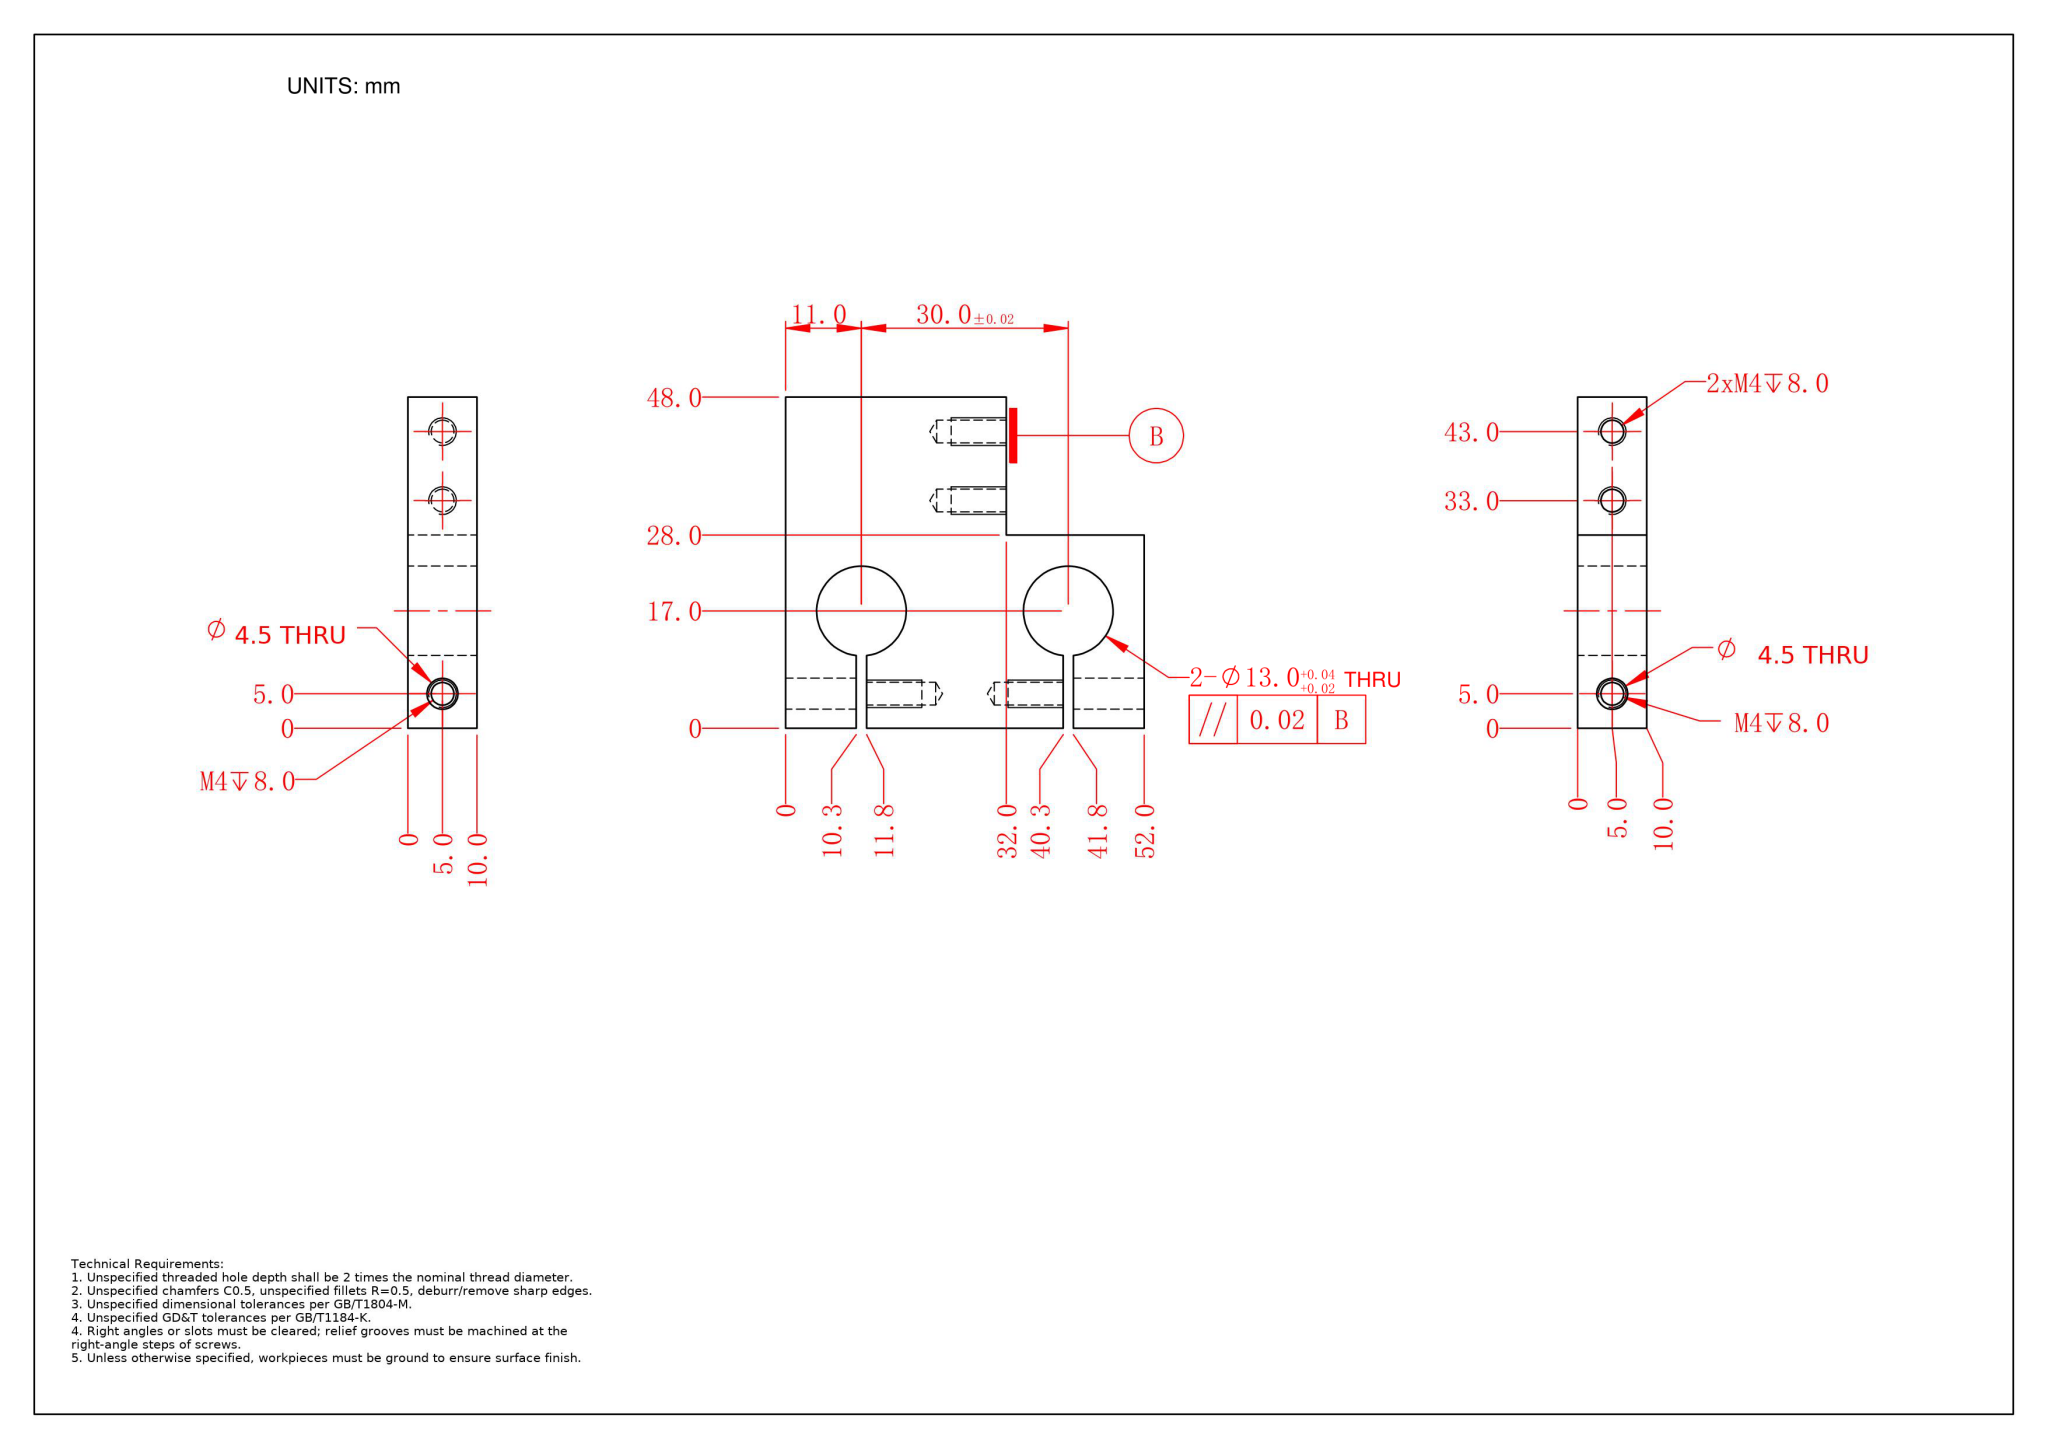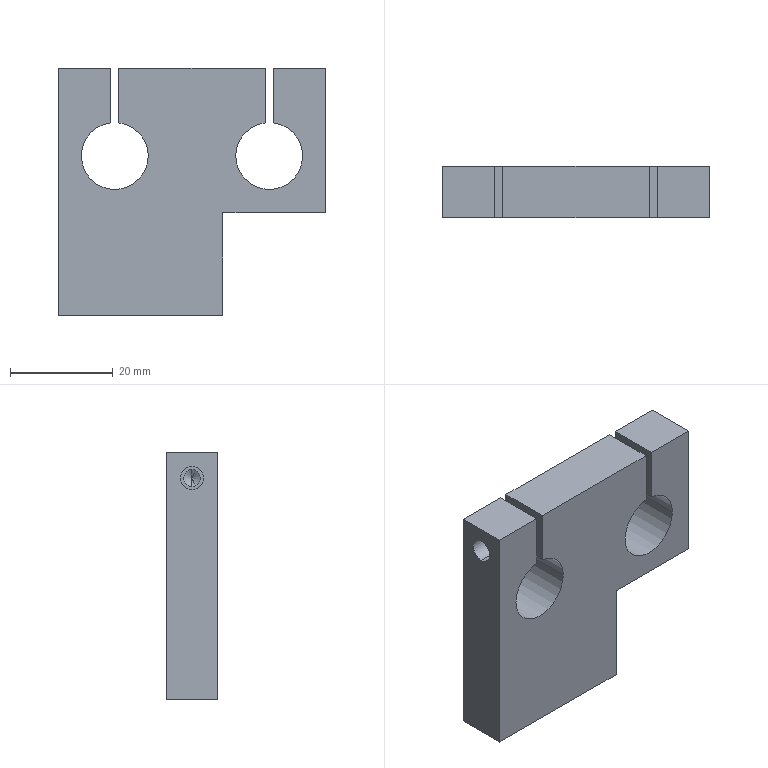Part | NX | mm | 1 solid | 40 faces | box 52 x 10 x 48 mm | volume 17309 mm3 | cylinder 18 | plane 14 | cone 8 | commonest cylinder face diameters 3.3 x8 13 x6 4.5 x4